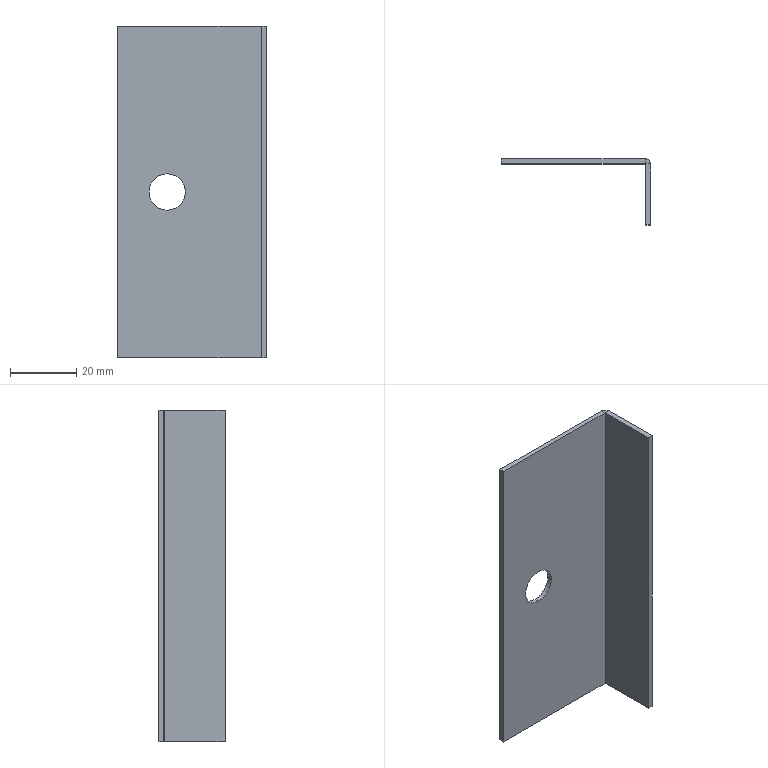Component | SolidWorks | LightBox-1_LightBoxBracket-1 | 1 solid | 16 faces | box 45 x 20 x 100 mm | volume 9328 mm3 | plane 12 | cylinder 4 | commonest cylinder face diameters 11 x2 3.2 x1 0.2 x1
STEP:
#1=COLOUR_RGB('',0.7922,0.8196,0.9333);
#2=FILL_AREA_STYLE_COLOUR('',#1);
#3=FILL_AREA_STYLE('',(#2));
#4=SURFACE_STYLE_FILL_AREA(#3);
#5=SURFACE_SIDE_STYLE('',(#4));
#6=SURFACE_STYLE_USAGE(.BOTH.,#5);
#7=PRESENTATION_STYLE_ASSIGNMENT((#6));
#8=CARTESIAN_POINT('',(-8.735,1.119,2.933));
#9=VERTEX_POINT('',#8);
#10=CARTESIAN_POINT('',(-8.735,1.119,3.366));
#11=VERTEX_POINT('',#10);
#12=CARTESIAN_POINT('',(-8.735,1.119,3.15));
#13=DIRECTION('',(0.,1.,0.));
#14=DIRECTION('',(0.,0.,1.));
#15=AXIS2_PLACEMENT_3D('',#12,#13,#14);
#16=CIRCLE('',#15,0.2165);
#17=EDGE_CURVE('',#9,#11,#16,.T.);
#18=ORIENTED_EDGE('',*,*,#17,.F.);
#19=CARTESIAN_POINT('',(-8.735,1.178,2.933));
#20=VERTEX_POINT('',#19);
#21=CARTESIAN_POINT('',(-8.735,1.119,2.933));
#22=DIRECTION('',(0.,1.,0.));
#23=VECTOR('',#22,39.37);
#24=LINE('',#21,#23);
#25=EDGE_CURVE('',#9,#20,#24,.T.);
#26=ORIENTED_EDGE('',*,*,#25,.T.);
#27=CARTESIAN_POINT('',(-8.735,1.178,3.366));
#28=VERTEX_POINT('',#27);
#29=CARTESIAN_POINT('',(-8.735,1.178,3.15));
#30=DIRECTION('',(0.,1.,0.));
#31=DIRECTION('',(0.,0.,1.));
#32=AXIS2_PLACEMENT_3D('',#29,#30,#31);
#33=CIRCLE('',#32,0.2165);
#34=EDGE_CURVE('',#20,#28,#33,.T.);
#35=ORIENTED_EDGE('',*,*,#34,.T.);
#36=CARTESIAN_POINT('',(-8.735,1.119,3.366));
#37=DIRECTION('',(0.,1.,0.));
#38=VECTOR('',#37,39.37);
#39=LINE('',#36,#38);
#40=EDGE_CURVE('',#11,#28,#39,.T.);
#41=ORIENTED_EDGE('',*,*,#40,.F.);
#42=EDGE_LOOP('',(#18,#26,#35,#41));
#43=FACE_OUTER_BOUND('',#42,.T.);
#44=CARTESIAN_POINT('',(-8.735,1.119,3.15));
#45=DIRECTION('',(0.,1.,0.));
#46=DIRECTION('',(0.,0.,1.));
#47=AXIS2_PLACEMENT_3D('',#44,#45,#46);
#48=CYLINDRICAL_SURFACE('',#47,0.2165);
#49=ADVANCED_FACE('',(#43),#48,.F.);
#50=CARTESIAN_POINT('',(-9.325,1.119,5.118));
#51=VERTEX_POINT('',#50);
#52=CARTESIAN_POINT('',(-7.617,1.119,5.118));
#53=VERTEX_POINT('',#52);
#54=CARTESIAN_POINT('',(-9.325,1.119,5.118));
#55=DIRECTION('',(1.,0.,0.));
#56=VECTOR('',#55,39.37);
#57=LINE('',#54,#56);
#58=EDGE_CURVE('',#51,#53,#57,.T.);
#59=ORIENTED_EDGE('',*,*,#58,.T.);
#60=CARTESIAN_POINT('',(-7.617,1.178,5.118));
#61=VERTEX_POINT('',#60);
#62=CARTESIAN_POINT('',(-7.617,1.119,5.118));
#63=DIRECTION('',(0.,1.,0.));
#64=VECTOR('',#63,39.37);
#65=LINE('',#62,#64);
#66=EDGE_CURVE('',#53,#61,#65,.T.);
#67=ORIENTED_EDGE('',*,*,#66,.T.);
#68=CARTESIAN_POINT('',(-9.325,1.178,5.118));
#69=VERTEX_POINT('',#68);
#70=CARTESIAN_POINT('',(-9.325,1.178,5.118));
#71=DIRECTION('',(1.,0.,0.));
#72=VECTOR('',#71,39.37);
#73=LINE('',#70,#72);
#74=EDGE_CURVE('',#69,#61,#73,.T.);
#75=ORIENTED_EDGE('',*,*,#74,.F.);
#76=CARTESIAN_POINT('',(-9.325,1.119,5.118));
#77=DIRECTION('',(0.,1.,0.));
#78=VECTOR('',#77,39.37);
#79=LINE('',#76,#78);
#80=EDGE_CURVE('',#51,#69,#79,.T.);
#81=ORIENTED_EDGE('',*,*,#80,.F.);
#82=EDGE_LOOP('',(#59,#67,#75,#81));
#83=FACE_OUTER_BOUND('',#82,.T.);
#84=CARTESIAN_POINT('',(-9.325,1.119,5.118));
#85=DIRECTION('',(0.,0.,1.));
#86=DIRECTION('',(1.,0.,0.));
#87=AXIS2_PLACEMENT_3D('',#84,#85,#86);
#88=PLANE('',#87);
#89=ADVANCED_FACE('',(#83),#88,.T.);
#90=CARTESIAN_POINT('',(-8.735,1.119,3.15));
#91=DIRECTION('',(0.,1.,0.));
#92=DIRECTION('',(0.,0.,1.));
#93=AXIS2_PLACEMENT_3D('',#90,#91,#92);
#94=CIRCLE('',#93,0.2165);
#95=EDGE_CURVE('',#11,#9,#94,.T.);
#96=ORIENTED_EDGE('',*,*,#95,.T.);
#97=ORIENTED_EDGE('',*,*,#17,.T.);
#98=EDGE_LOOP('',(#96,#97));
#99=FACE_BOUND('',#98,.T.);
#100=CARTESIAN_POINT('',(-7.617,1.119,1.181));
#101=VERTEX_POINT('',#100);
#102=CARTESIAN_POINT('',(-9.325,1.119,1.181));
#103=VERTEX_POINT('',#102);
#104=CARTESIAN_POINT('',(-9.325,1.119,1.181));
#105=DIRECTION('',(-1.,0.,0.));
#106=VECTOR('',#105,39.37);
#107=LINE('',#104,#106);
#108=EDGE_CURVE('',#101,#103,#107,.T.);
#109=ORIENTED_EDGE('',*,*,#108,.F.);
#110=CARTESIAN_POINT('',(-7.617,1.119,5.118));
#111=DIRECTION('',(0.,0.,-1.));
#112=VECTOR('',#111,39.37);
#113=LINE('',#110,#112);
#114=EDGE_CURVE('',#53,#101,#113,.T.);
#115=ORIENTED_EDGE('',*,*,#114,.F.);
#116=ORIENTED_EDGE('',*,*,#58,.F.);
#117=CARTESIAN_POINT('',(-9.325,1.119,5.118));
#118=DIRECTION('',(0.,0.,1.));
#119=VECTOR('',#118,39.37);
#120=LINE('',#117,#119);
#121=EDGE_CURVE('',#103,#51,#120,.T.);
#122=ORIENTED_EDGE('',*,*,#121,.F.);
#123=EDGE_LOOP('',(#109,#115,#116,#122));
#124=FACE_OUTER_BOUND('',#123,.T.);
#125=CARTESIAN_POINT('',(-9.671,1.119,3.618));
#126=DIRECTION('',(0.,-1.,0.));
#127=DIRECTION('',(0.,0.,-1.));
#128=AXIS2_PLACEMENT_3D('',#125,#126,#127);
#129=PLANE('',#128);
#130=ADVANCED_FACE('',(#99,#124),#129,.T.);
#131=CARTESIAN_POINT('',(-8.735,1.178,3.15));
#132=DIRECTION('',(0.,1.,0.));
#133=DIRECTION('',(0.,0.,1.));
#134=AXIS2_PLACEMENT_3D('',#131,#132,#133);
#135=CIRCLE('',#134,0.2165);
#136=EDGE_CURVE('',#28,#20,#135,.T.);
#137=ORIENTED_EDGE('',*,*,#136,.F.);
#138=ORIENTED_EDGE('',*,*,#34,.F.);
#139=EDGE_LOOP('',(#137,#138));
#140=FACE_BOUND('',#139,.T.);
#141=CARTESIAN_POINT('',(-7.617,1.178,1.181));
#142=VERTEX_POINT('',#141);
#143=CARTESIAN_POINT('',(-7.617,1.178,5.118));
#144=DIRECTION('',(0.,0.,-1.));
#145=VECTOR('',#144,39.37);
#146=LINE('',#143,#145);
#147=EDGE_CURVE('',#61,#142,#146,.T.);
#148=ORIENTED_EDGE('',*,*,#147,.T.);
#149=CARTESIAN_POINT('',(-9.325,1.178,1.181));
#150=VERTEX_POINT('',#149);
#151=CARTESIAN_POINT('',(-9.325,1.178,1.181));
#152=DIRECTION('',(-1.,0.,0.));
#153=VECTOR('',#152,39.37);
#154=LINE('',#151,#153);
#155=EDGE_CURVE('',#142,#150,#154,.T.);
#156=ORIENTED_EDGE('',*,*,#155,.T.);
#157=CARTESIAN_POINT('',(-9.325,1.178,5.118));
#158=DIRECTION('',(0.,0.,1.));
#159=VECTOR('',#158,39.37);
#160=LINE('',#157,#159);
#161=EDGE_CURVE('',#150,#69,#160,.T.);
#162=ORIENTED_EDGE('',*,*,#161,.T.);
#163=ORIENTED_EDGE('',*,*,#74,.T.);
#164=EDGE_LOOP('',(#148,#156,#162,#163));
#165=FACE_OUTER_BOUND('',#164,.T.);
#166=CARTESIAN_POINT('',(-9.671,1.178,3.618));
#167=DIRECTION('',(0.,-1.,0.));
#168=DIRECTION('',(0.,0.,-1.));
#169=AXIS2_PLACEMENT_3D('',#166,#167,#168);
#170=PLANE('',#169);
#171=ADVANCED_FACE('',(#140,#165),#170,.F.);
#172=ORIENTED_EDGE('',*,*,#161,.F.);
#173=CARTESIAN_POINT('',(-9.325,1.119,1.181));
#174=DIRECTION('',(0.,1.,0.));
#175=VECTOR('',#174,39.37);
#176=LINE('',#173,#175);
#177=EDGE_CURVE('',#103,#150,#176,.T.);
#178=ORIENTED_EDGE('',*,*,#177,.F.);
#179=ORIENTED_EDGE('',*,*,#121,.T.);
#180=ORIENTED_EDGE('',*,*,#80,.T.);
#181=EDGE_LOOP('',(#172,#178,#179,#180));
#182=FACE_OUTER_BOUND('',#181,.T.);
#183=CARTESIAN_POINT('',(-9.325,1.119,5.118));
#184=DIRECTION('',(-1.,0.,0.));
#185=DIRECTION('',(0.,0.,1.));
#186=AXIS2_PLACEMENT_3D('',#183,#184,#185);
#187=PLANE('',#186);
#188=ADVANCED_FACE('',(#182),#187,.T.);
#189=CARTESIAN_POINT('',(-7.617,1.119,1.181));
#190=DIRECTION('',(0.,1.,0.));
#191=VECTOR('',#190,39.37);
#192=LINE('',#189,#191);
#193=EDGE_CURVE('',#101,#142,#192,.T.);
#194=ORIENTED_EDGE('',*,*,#193,.F.);
#195=ORIENTED_EDGE('',*,*,#108,.T.);
#196=ORIENTED_EDGE('',*,*,#177,.T.);
#197=ORIENTED_EDGE('',*,*,#155,.F.);
#198=EDGE_LOOP('',(#194,#195,#196,#197));
#199=FACE_OUTER_BOUND('',#198,.T.);
#200=CARTESIAN_POINT('',(-9.325,1.119,1.181));
#201=DIRECTION('',(0.,0.,-1.));
#202=DIRECTION('',(-1.,0.,0.));
#203=AXIS2_PLACEMENT_3D('',#200,#201,#202);
#204=PLANE('',#203);
#205=ADVANCED_FACE('',(#199),#204,.T.);
#206=ORIENTED_EDGE('',*,*,#25,.F.);
#207=ORIENTED_EDGE('',*,*,#95,.F.);
#208=ORIENTED_EDGE('',*,*,#40,.T.);
#209=ORIENTED_EDGE('',*,*,#136,.T.);
#210=EDGE_LOOP('',(#206,#207,#208,#209));
#211=FACE_OUTER_BOUND('',#210,.T.);
#212=CARTESIAN_POINT('',(-8.735,1.119,3.15));
#213=DIRECTION('',(0.,1.,0.));
#214=DIRECTION('',(0.,0.,1.));
#215=AXIS2_PLACEMENT_3D('',#212,#213,#214);
#216=CYLINDRICAL_SURFACE('',#215,0.2165);
#217=ADVANCED_FACE('',(#211),#216,.F.);
#218=CARTESIAN_POINT('',(-7.613,1.115,1.181));
#219=VERTEX_POINT('',#218);
#220=CARTESIAN_POINT('',(-7.554,1.115,1.181));
#221=VERTEX_POINT('',#220);
#222=CARTESIAN_POINT('',(-7.554,1.115,1.181));
#223=DIRECTION('',(1.,0.,0.));
#224=VECTOR('',#223,39.37);
#225=LINE('',#222,#224);
#226=EDGE_CURVE('',#219,#221,#225,.T.);
#227=ORIENTED_EDGE('',*,*,#226,.F.);
#228=CARTESIAN_POINT('',(-7.617,1.115,1.181));
#229=DIRECTION('',(0.,0.,-1.));
#230=DIRECTION('',(1.,0.,0.));
#231=AXIS2_PLACEMENT_3D('',#228,#229,#230);
#232=CIRCLE('',#231,0.003937);
#233=EDGE_CURVE('',#101,#219,#232,.T.);
#234=ORIENTED_EDGE('',*,*,#233,.F.);
#235=ORIENTED_EDGE('',*,*,#193,.T.);
#236=CARTESIAN_POINT('',(-7.617,1.115,1.181));
#237=DIRECTION('',(0.,0.,-1.));
#238=DIRECTION('',(1.,-0.,0.));
#239=AXIS2_PLACEMENT_3D('',#236,#237,#238);
#240=CIRCLE('',#239,0.06299);
#241=EDGE_CURVE('',#142,#221,#240,.T.);
#242=ORIENTED_EDGE('',*,*,#241,.T.);
#243=EDGE_LOOP('',(#227,#234,#235,#242));
#244=FACE_OUTER_BOUND('',#243,.T.);
#245=CARTESIAN_POINT('',(-7.617,1.115,1.181));
#246=DIRECTION('',(0.,0.,-1.));
#247=DIRECTION('',(-1.,0.,0.));
#248=AXIS2_PLACEMENT_3D('',#245,#246,#247);
#249=PLANE('',#248);
#250=ADVANCED_FACE('',(#244),#249,.T.);
#251=CARTESIAN_POINT('',(-7.613,1.115,5.118));
#252=VERTEX_POINT('',#251);
#253=CARTESIAN_POINT('',(-7.617,1.115,5.118));
#254=DIRECTION('',(0.,0.,1.));
#255=DIRECTION('',(1.,0.,0.));
#256=AXIS2_PLACEMENT_3D('',#253,#254,#255);
#257=CIRCLE('',#256,0.003937);
#258=EDGE_CURVE('',#252,#53,#257,.T.);
#259=ORIENTED_EDGE('',*,*,#258,.F.);
#260=CARTESIAN_POINT('',(-7.554,1.115,5.118));
#261=VERTEX_POINT('',#260);
#262=CARTESIAN_POINT('',(-7.613,1.115,5.118));
#263=DIRECTION('',(1.,0.,0.));
#264=VECTOR('',#263,39.37);
#265=LINE('',#262,#264);
#266=EDGE_CURVE('',#252,#261,#265,.T.);
#267=ORIENTED_EDGE('',*,*,#266,.T.);
#268=CARTESIAN_POINT('',(-7.617,1.115,5.118));
#269=DIRECTION('',(0.,0.,1.));
#270=DIRECTION('',(1.,0.,0.));
#271=AXIS2_PLACEMENT_3D('',#268,#269,#270);
#272=CIRCLE('',#271,0.06299);
#273=EDGE_CURVE('',#261,#61,#272,.T.);
#274=ORIENTED_EDGE('',*,*,#273,.T.);
#275=ORIENTED_EDGE('',*,*,#66,.F.);
#276=EDGE_LOOP('',(#259,#267,#274,#275));
#277=FACE_OUTER_BOUND('',#276,.T.);
#278=CARTESIAN_POINT('',(-7.617,1.115,5.118));
#279=DIRECTION('',(0.,0.,-1.));
#280=DIRECTION('',(-1.,0.,0.));
#281=AXIS2_PLACEMENT_3D('',#278,#279,#280);
#282=PLANE('',#281);
#283=ADVANCED_FACE('',(#277),#282,.F.);
#284=ORIENTED_EDGE('',*,*,#147,.F.);
#285=ORIENTED_EDGE('',*,*,#273,.F.);
#286=CARTESIAN_POINT('',(-7.554,1.115,3.618));
#287=DIRECTION('',(0.,0.,1.));
#288=VECTOR('',#287,39.37);
#289=LINE('',#286,#288);
#290=EDGE_CURVE('',#221,#261,#289,.T.);
#291=ORIENTED_EDGE('',*,*,#290,.F.);
#292=ORIENTED_EDGE('',*,*,#241,.F.);
#293=EDGE_LOOP('',(#284,#285,#291,#292));
#294=FACE_OUTER_BOUND('',#293,.T.);
#295=CARTESIAN_POINT('',(-7.617,1.115,5.118));
#296=DIRECTION('',(0.,0.,1.));
#297=DIRECTION('',(1.,0.,0.));
#298=AXIS2_PLACEMENT_3D('',#295,#296,#297);
#299=CYLINDRICAL_SURFACE('',#298,0.06299);
#300=ADVANCED_FACE('',(#294),#299,.T.);
#301=ORIENTED_EDGE('',*,*,#114,.T.);
#302=ORIENTED_EDGE('',*,*,#233,.T.);
#303=CARTESIAN_POINT('',(-7.613,1.115,1.181));
#304=DIRECTION('',(0.,0.,1.));
#305=VECTOR('',#304,39.37);
#306=LINE('',#303,#305);
#307=EDGE_CURVE('',#219,#252,#306,.T.);
#308=ORIENTED_EDGE('',*,*,#307,.T.);
#309=ORIENTED_EDGE('',*,*,#258,.T.);
#310=EDGE_LOOP('',(#301,#302,#308,#309));
#311=FACE_OUTER_BOUND('',#310,.T.);
#312=CARTESIAN_POINT('',(-7.617,1.115,5.118));
#313=DIRECTION('',(0.,0.,1.));
#314=DIRECTION('',(1.,0.,0.));
#315=AXIS2_PLACEMENT_3D('',#312,#313,#314);
#316=CYLINDRICAL_SURFACE('',#315,0.003937);
#317=ADVANCED_FACE('',(#311),#316,.F.);
#318=CARTESIAN_POINT('',(-7.554,0.3903,5.118));
#319=VERTEX_POINT('',#318);
#320=CARTESIAN_POINT('',(-7.554,1.119,5.118));
#321=DIRECTION('',(-0.,1.,0.));
#322=VECTOR('',#321,39.37);
#323=LINE('',#320,#322);
#324=EDGE_CURVE('',#319,#261,#323,.T.);
#325=ORIENTED_EDGE('',*,*,#324,.T.);
#326=ORIENTED_EDGE('',*,*,#266,.F.);
#327=CARTESIAN_POINT('',(-7.613,0.3903,5.118));
#328=VERTEX_POINT('',#327);
#329=CARTESIAN_POINT('',(-7.613,1.178,5.118));
#330=DIRECTION('',(-0.,1.,0.));
#331=VECTOR('',#330,39.37);
#332=LINE('',#329,#331);
#333=EDGE_CURVE('',#328,#252,#332,.T.);
#334=ORIENTED_EDGE('',*,*,#333,.F.);
#335=CARTESIAN_POINT('',(-7.554,0.3903,5.118));
#336=DIRECTION('',(-1.,-0.,0.));
#337=VECTOR('',#336,39.37);
#338=LINE('',#335,#337);
#339=EDGE_CURVE('',#319,#328,#338,.T.);
#340=ORIENTED_EDGE('',*,*,#339,.F.);
#341=EDGE_LOOP('',(#325,#326,#334,#340));
#342=FACE_OUTER_BOUND('',#341,.T.);
#343=CARTESIAN_POINT('',(-7.554,1.119,5.118));
#344=DIRECTION('',(0.,0.,1.));
#345=DIRECTION('',(1.,0.,0.));
#346=AXIS2_PLACEMENT_3D('',#343,#344,#345);
#347=PLANE('',#346);
#348=ADVANCED_FACE('',(#342),#347,.T.);
#349=CARTESIAN_POINT('',(-7.613,0.3903,1.181));
#350=VERTEX_POINT('',#349);
#351=CARTESIAN_POINT('',(-7.613,1.178,1.181));
#352=DIRECTION('',(0.,-1.,0.));
#353=VECTOR('',#352,39.37);
#354=LINE('',#351,#353);
#355=EDGE_CURVE('',#219,#350,#354,.T.);
#356=ORIENTED_EDGE('',*,*,#355,.F.);
#357=ORIENTED_EDGE('',*,*,#226,.T.);
#358=CARTESIAN_POINT('',(-7.554,0.3903,1.181));
#359=VERTEX_POINT('',#358);
#360=CARTESIAN_POINT('',(-7.554,0.3903,1.181));
#361=DIRECTION('',(0.,-1.,0.));
#362=VECTOR('',#361,39.37);
#363=LINE('',#360,#362);
#364=EDGE_CURVE('',#221,#359,#363,.T.);
#365=ORIENTED_EDGE('',*,*,#364,.T.);
#366=CARTESIAN_POINT('',(-7.554,0.3903,1.181));
#367=DIRECTION('',(-1.,-0.,0.));
#368=VECTOR('',#367,39.37);
#369=LINE('',#366,#368);
#370=EDGE_CURVE('',#359,#350,#369,.T.);
#371=ORIENTED_EDGE('',*,*,#370,.T.);
#372=EDGE_LOOP('',(#356,#357,#365,#371));
#373=FACE_OUTER_BOUND('',#372,.T.);
#374=CARTESIAN_POINT('',(-7.554,0.3903,1.181));
#375=DIRECTION('',(0.,0.,-1.));
#376=DIRECTION('',(-1.,0.,0.));
#377=AXIS2_PLACEMENT_3D('',#374,#375,#376);
#378=PLANE('',#377);
#379=ADVANCED_FACE('',(#373),#378,.T.);
#380=ORIENTED_EDGE('',*,*,#364,.F.);
#381=ORIENTED_EDGE('',*,*,#290,.T.);
#382=ORIENTED_EDGE('',*,*,#324,.F.);
#383=CARTESIAN_POINT('',(-7.554,0.3903,5.118));
#384=DIRECTION('',(0.,0.,1.));
#385=VECTOR('',#384,39.37);
#386=LINE('',#383,#385);
#387=EDGE_CURVE('',#359,#319,#386,.T.);
#388=ORIENTED_EDGE('',*,*,#387,.F.);
#389=EDGE_LOOP('',(#380,#381,#382,#388));
#390=FACE_OUTER_BOUND('',#389,.T.);
#391=CARTESIAN_POINT('',(-7.554,1.178,3.618));
#392=DIRECTION('',(1.,0.,0.));
#393=DIRECTION('',(-0.,1.,0.));
#394=AXIS2_PLACEMENT_3D('',#391,#392,#393);
#395=PLANE('',#394);
#396=ADVANCED_FACE('',(#390),#395,.T.);
#397=ORIENTED_EDGE('',*,*,#307,.F.);
#398=ORIENTED_EDGE('',*,*,#355,.T.);
#399=CARTESIAN_POINT('',(-7.613,0.3903,3.618));
#400=DIRECTION('',(0.,0.,1.));
#401=VECTOR('',#400,39.37);
#402=LINE('',#399,#401);
#403=EDGE_CURVE('',#350,#328,#402,.T.);
#404=ORIENTED_EDGE('',*,*,#403,.T.);
#405=ORIENTED_EDGE('',*,*,#333,.T.);
#406=EDGE_LOOP('',(#397,#398,#404,#405));
#407=FACE_OUTER_BOUND('',#406,.T.);
#408=CARTESIAN_POINT('',(-7.613,1.178,3.618));
#409=DIRECTION('',(1.,0.,0.));
#410=DIRECTION('',(-0.,1.,0.));
#411=AXIS2_PLACEMENT_3D('',#408,#409,#410);
#412=PLANE('',#411);
#413=ADVANCED_FACE('',(#407),#412,.F.);
#414=ORIENTED_EDGE('',*,*,#403,.F.);
#415=ORIENTED_EDGE('',*,*,#370,.F.);
#416=ORIENTED_EDGE('',*,*,#387,.T.);
#417=ORIENTED_EDGE('',*,*,#339,.T.);
#418=EDGE_LOOP('',(#414,#415,#416,#417));
#419=FACE_OUTER_BOUND('',#418,.T.);
#420=CARTESIAN_POINT('',(-7.554,0.3903,5.118));
#421=DIRECTION('',(0.,-1.,0.));
#422=DIRECTION('',(1.,0.,0.));
#423=AXIS2_PLACEMENT_3D('',#420,#421,#422);
#424=PLANE('',#423);
#425=ADVANCED_FACE('',(#419),#424,.T.);
#426=CLOSED_SHELL('',(#49,#89,#130,#171,#188,#205,#217,#250,#283,#300,#317,#348,#379,#396,#413,#425));
#427=MANIFOLD_SOLID_BREP('',#426);
#428=STYLED_ITEM('',(#7),#427);
#429=PRESENTATION_LAYER_ASSIGNMENT('','',(#428));
#430=CARTESIAN_POINT('',(0.,0.,0.));
#431=DIRECTION('',(0.,0.,1.));
#432=DIRECTION('',(1.,0.,0.));
#433=AXIS2_PLACEMENT_3D('',#430,#431,#432);
#434=(LENGTH_UNIT()NAMED_UNIT(*)SI_UNIT($,.METRE.));
#435=LENGTH_MEASURE_WITH_UNIT(LENGTH_MEASURE(0.0254),#434);
#436=DIMENSIONAL_EXPONENTS(1.,0.,0.,0.,0.,0.,0.);
#437=(CONVERSION_BASED_UNIT('',#435)LENGTH_UNIT()NAMED_UNIT(#436));
#438=UNCERTAINTY_MEASURE_WITH_UNIT(LENGTH_MEASURE(0.00001),#437,'','');
#439=(NAMED_UNIT(*)PLANE_ANGLE_UNIT()SI_UNIT($,.RADIAN.));
#440=(NAMED_UNIT(*)SI_UNIT($,.STERADIAN.)SOLID_ANGLE_UNIT());
#441=(GEOMETRIC_REPRESENTATION_CONTEXT(3)GLOBAL_UNCERTAINTY_ASSIGNED_CONTEXT((#438))GLOBAL_UNIT_ASSIGNED_CONTEXT((#437,#439,#440))REPRESENTATION_CONTEXT('',''));
#442=ADVANCED_BREP_SHAPE_REPRESENTATION('',(#427,#433),#441);
#443=(LENGTH_UNIT()NAMED_UNIT(*)SI_UNIT($,.METRE.));
#444=LENGTH_MEASURE_WITH_UNIT(LENGTH_MEASURE(0.0254),#443);
#445=DIMENSIONAL_EXPONENTS(1.,0.,0.,0.,0.,0.,0.);
#446=(CONVERSION_BASED_UNIT('',#444)LENGTH_UNIT()NAMED_UNIT(#445));
#447=UNCERTAINTY_MEASURE_WITH_UNIT(LENGTH_MEASURE(0.00001),#446,'','');
#448=(NAMED_UNIT(*)PLANE_ANGLE_UNIT()SI_UNIT($,.RADIAN.));
#449=(NAMED_UNIT(*)SI_UNIT($,.STERADIAN.)SOLID_ANGLE_UNIT());
#450=(GEOMETRIC_REPRESENTATION_CONTEXT(3)GLOBAL_UNCERTAINTY_ASSIGNED_CONTEXT((#447))GLOBAL_UNIT_ASSIGNED_CONTEXT((#446,#448,#449))REPRESENTATION_CONTEXT('',''));
#451=MECHANICAL_DESIGN_GEOMETRIC_PRESENTATION_REPRESENTATION('',(#428),#450);